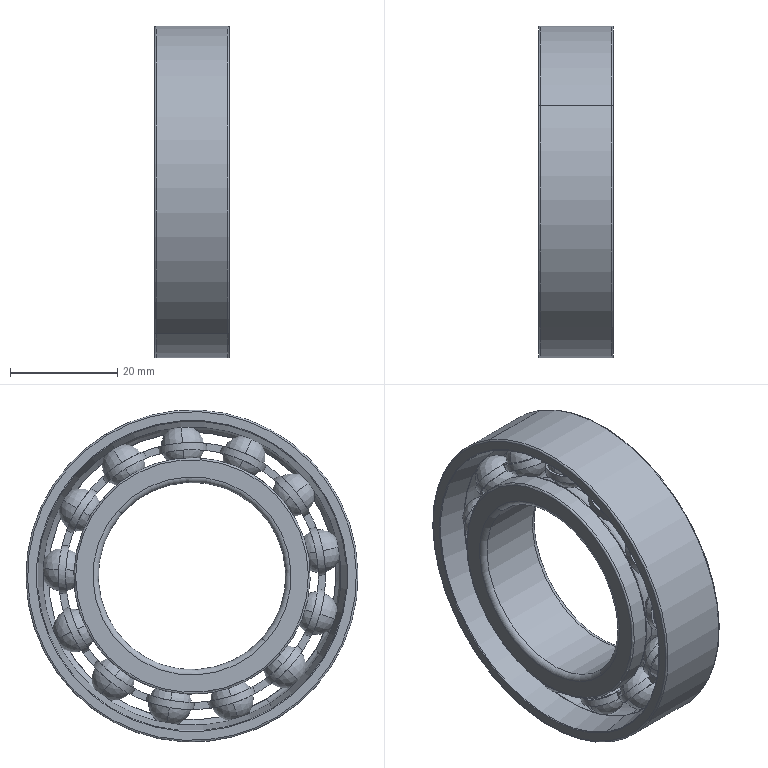Component | SolidWorks | 2-10-10WorkpieceAxisAssembly-1_2-10-8Bearing7007AC-2 | 16 solids | 156 faces | volume 18750 mm3 | cylinder 66 | torus 32 | plane 30 | sphere 26 | cone 2 | commonest cylinder face diameters 8.017 x26 8.979 x26 44.138 x4 35 x2 53.692 x2 62 x2 47.164 x2 49.836 x2